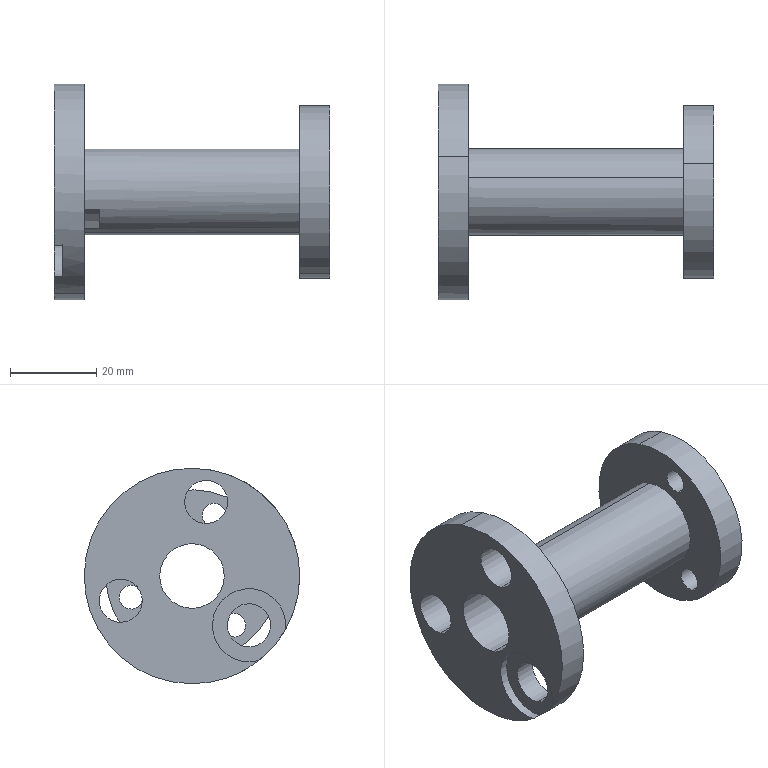Component | SolidWorks | SuctionCupBracket-1 | 1 solid | 29 faces | box 64 x 50 x 50 mm | volume 24493 mm3 | cylinder 23 | plane 6 | commonest cylinder face diameters 10 x6 5.5 x6 17 x3 15 x2 50 x2 40 x2 20 x2
STEP:
#1=COLOUR_RGB('',0.7922,0.8196,0.9333);
#2=FILL_AREA_STYLE_COLOUR('',#1);
#3=FILL_AREA_STYLE('',(#2));
#4=SURFACE_STYLE_FILL_AREA(#3);
#5=SURFACE_SIDE_STYLE('',(#4));
#6=SURFACE_STYLE_USAGE(.BOTH.,#5);
#7=PRESENTATION_STYLE_ASSIGNMENT((#6));
#8=CARTESIAN_POINT('',(-5.854,1.572,-3.839));
#9=VERTEX_POINT('',#8);
#10=CARTESIAN_POINT('',(-5.854,1.375,-4.478));
#11=VERTEX_POINT('',#10);
#12=CARTESIAN_POINT('',(-5.854,1.462,-4.155));
#13=DIRECTION('',(-1.,0.,0.));
#14=DIRECTION('',(0.,0.3282,0.9446));
#15=AXIS2_PLACEMENT_3D('',#12,#13,#14);
#16=CIRCLE('',#15,0.3346);
#17=EDGE_CURVE('',#9,#11,#16,.T.);
#18=ORIENTED_EDGE('',*,*,#17,.F.);
#19=CARTESIAN_POINT('',(-5.933,1.572,-3.839));
#20=VERTEX_POINT('',#19);
#21=CARTESIAN_POINT('',(-5.854,1.572,-3.839));
#22=DIRECTION('',(-1.,0.,0.));
#23=VECTOR('',#22,39.37);
#24=LINE('',#21,#23);
#25=EDGE_CURVE('',#9,#20,#24,.T.);
#26=ORIENTED_EDGE('',*,*,#25,.T.);
#27=CARTESIAN_POINT('',(-5.933,1.375,-4.478));
#28=VERTEX_POINT('',#27);
#29=CARTESIAN_POINT('',(-5.933,1.462,-4.155));
#30=DIRECTION('',(-1.,0.,0.));
#31=DIRECTION('',(0.,0.3282,0.9446));
#32=AXIS2_PLACEMENT_3D('',#29,#30,#31);
#33=CIRCLE('',#32,0.3346);
#34=EDGE_CURVE('',#20,#28,#33,.T.);
#35=ORIENTED_EDGE('',*,*,#34,.T.);
#36=CARTESIAN_POINT('',(-5.893,1.375,-4.478));
#37=DIRECTION('',(-1.,0.,0.));
#38=VECTOR('',#37,39.37);
#39=LINE('',#36,#38);
#40=EDGE_CURVE('',#11,#28,#39,.T.);
#41=ORIENTED_EDGE('',*,*,#40,.F.);
#42=EDGE_LOOP('',(#18,#26,#35,#41));
#43=FACE_OUTER_BOUND('',#42,.T.);
#44=CARTESIAN_POINT('',(-5.854,1.462,-4.155));
#45=DIRECTION('',(-1.,0.,0.));
#46=DIRECTION('',(0.,0.3282,0.9446));
#47=AXIS2_PLACEMENT_3D('',#44,#45,#46);
#48=CYLINDRICAL_SURFACE('',#47,0.3346);
#49=ADVANCED_FACE('',(#43),#48,.F.);
#50=CARTESIAN_POINT('',(-5.657,1.789,-3.214));
#51=VERTEX_POINT('',#50);
#52=CARTESIAN_POINT('',(-5.657,1.919,-2.842));
#53=VERTEX_POINT('',#52);
#54=CARTESIAN_POINT('',(-5.657,1.854,-3.028));
#55=DIRECTION('',(-1.,0.,0.));
#56=DIRECTION('',(0.,-0.9822,-0.1881));
#57=AXIS2_PLACEMENT_3D('',#54,#55,#56);
#58=CIRCLE('',#57,0.1969);
#59=EDGE_CURVE('',#51,#53,#58,.T.);
#60=ORIENTED_EDGE('',*,*,#59,.F.);
#61=CARTESIAN_POINT('',(-5.933,1.789,-3.214));
#62=VERTEX_POINT('',#61);
#63=CARTESIAN_POINT('',(-5.657,1.789,-3.214));
#64=DIRECTION('',(-1.,0.,0.));
#65=VECTOR('',#64,39.37);
#66=LINE('',#63,#65);
#67=EDGE_CURVE('',#51,#62,#66,.T.);
#68=ORIENTED_EDGE('',*,*,#67,.T.);
#69=CARTESIAN_POINT('',(-5.933,1.919,-2.842));
#70=VERTEX_POINT('',#69);
#71=CARTESIAN_POINT('',(-5.933,1.854,-3.028));
#72=DIRECTION('',(-1.,0.,0.));
#73=DIRECTION('',(0.,-0.9822,-0.1881));
#74=AXIS2_PLACEMENT_3D('',#71,#72,#73);
#75=CIRCLE('',#74,0.1969);
#76=EDGE_CURVE('',#62,#70,#75,.T.);
#77=ORIENTED_EDGE('',*,*,#76,.T.);
#78=CARTESIAN_POINT('',(-5.657,1.919,-2.842));
#79=DIRECTION('',(-1.,0.,0.));
#80=VECTOR('',#79,39.37);
#81=LINE('',#78,#80);
#82=EDGE_CURVE('',#53,#70,#81,.T.);
#83=ORIENTED_EDGE('',*,*,#82,.F.);
#84=EDGE_LOOP('',(#60,#68,#77,#83));
#85=FACE_OUTER_BOUND('',#84,.T.);
#86=CARTESIAN_POINT('',(-5.657,1.854,-3.028));
#87=DIRECTION('',(-1.,0.,0.));
#88=DIRECTION('',(0.,0.3282,0.9446));
#89=AXIS2_PLACEMENT_3D('',#86,#87,#88);
#90=CYLINDRICAL_SURFACE('',#89,0.1969);
#91=ADVANCED_FACE('',(#85),#90,.F.);
#92=CARTESIAN_POINT('',(-5.657,2.57,-4.117));
#93=VERTEX_POINT('',#92);
#94=CARTESIAN_POINT('',(-5.657,2.699,-3.745));
#95=VERTEX_POINT('',#94);
#96=CARTESIAN_POINT('',(-5.657,2.634,-3.931));
#97=DIRECTION('',(-1.,0.,0.));
#98=DIRECTION('',(0.,0.3282,0.9446));
#99=AXIS2_PLACEMENT_3D('',#96,#97,#98);
#100=CIRCLE('',#99,0.1969);
#101=EDGE_CURVE('',#93,#95,#100,.T.);
#102=ORIENTED_EDGE('',*,*,#101,.F.);
#103=CARTESIAN_POINT('',(-5.933,2.57,-4.117));
#104=VERTEX_POINT('',#103);
#105=CARTESIAN_POINT('',(-5.657,2.57,-4.117));
#106=DIRECTION('',(-1.,0.,0.));
#107=VECTOR('',#106,39.37);
#108=LINE('',#105,#107);
#109=EDGE_CURVE('',#93,#104,#108,.T.);
#110=ORIENTED_EDGE('',*,*,#109,.T.);
#111=CARTESIAN_POINT('',(-5.933,2.699,-3.745));
#112=VERTEX_POINT('',#111);
#113=CARTESIAN_POINT('',(-5.933,2.634,-3.931));
#114=DIRECTION('',(-1.,0.,0.));
#115=DIRECTION('',(0.,0.3282,0.9446));
#116=AXIS2_PLACEMENT_3D('',#113,#114,#115);
#117=CIRCLE('',#116,0.1969);
#118=EDGE_CURVE('',#104,#112,#117,.T.);
#119=ORIENTED_EDGE('',*,*,#118,.T.);
#120=CARTESIAN_POINT('',(-5.657,2.699,-3.745));
#121=DIRECTION('',(-1.,0.,0.));
#122=VECTOR('',#121,39.37);
#123=LINE('',#120,#122);
#124=EDGE_CURVE('',#95,#112,#123,.T.);
#125=ORIENTED_EDGE('',*,*,#124,.F.);
#126=EDGE_LOOP('',(#102,#110,#119,#125));
#127=FACE_OUTER_BOUND('',#126,.T.);
#128=CARTESIAN_POINT('',(-5.657,2.634,-3.931));
#129=DIRECTION('',(-1.,0.,0.));
#130=DIRECTION('',(0.,0.3282,0.9446));
#131=AXIS2_PLACEMENT_3D('',#128,#129,#130);
#132=CYLINDRICAL_SURFACE('',#131,0.1969);
#133=ADVANCED_FACE('',(#127),#132,.F.);
#134=CARTESIAN_POINT('',(-5.933,2.08,-3.426));
#135=VERTEX_POINT('',#134);
#136=CARTESIAN_POINT('',(-5.933,1.887,-3.983));
#137=VERTEX_POINT('',#136);
#138=CARTESIAN_POINT('',(-5.933,1.983,-3.704));
#139=DIRECTION('',(1.,-0.,-0.));
#140=DIRECTION('',(0.,-0.3282,-0.9446));
#141=AXIS2_PLACEMENT_3D('',#138,#139,#140);
#142=CIRCLE('',#141,0.2953);
#143=EDGE_CURVE('',#135,#137,#142,.T.);
#144=ORIENTED_EDGE('',*,*,#143,.F.);
#145=CARTESIAN_POINT('',(-3.413,2.08,-3.426));
#146=VERTEX_POINT('',#145);
#147=CARTESIAN_POINT('',(-5.933,2.08,-3.426));
#148=DIRECTION('',(1.,-0.,-0.));
#149=VECTOR('',#148,39.37);
#150=LINE('',#147,#149);
#151=EDGE_CURVE('',#135,#146,#150,.T.);
#152=ORIENTED_EDGE('',*,*,#151,.T.);
#153=CARTESIAN_POINT('',(-3.413,1.887,-3.983));
#154=VERTEX_POINT('',#153);
#155=CARTESIAN_POINT('',(-3.413,1.983,-3.704));
#156=DIRECTION('',(1.,-0.,-0.));
#157=DIRECTION('',(0.,-0.3282,-0.9446));
#158=AXIS2_PLACEMENT_3D('',#155,#156,#157);
#159=CIRCLE('',#158,0.2953);
#160=EDGE_CURVE('',#146,#154,#159,.T.);
#161=ORIENTED_EDGE('',*,*,#160,.T.);
#162=CARTESIAN_POINT('',(-5.933,1.887,-3.983));
#163=DIRECTION('',(1.,-0.,-0.));
#164=VECTOR('',#163,39.37);
#165=LINE('',#162,#164);
#166=EDGE_CURVE('',#137,#154,#165,.T.);
#167=ORIENTED_EDGE('',*,*,#166,.F.);
#168=EDGE_LOOP('',(#144,#152,#161,#167));
#169=FACE_OUTER_BOUND('',#168,.T.);
#170=CARTESIAN_POINT('',(-5.933,1.983,-3.704));
#171=DIRECTION('',(1.,-0.,-0.));
#172=DIRECTION('',(0.,-0.3282,-0.9446));
#173=AXIS2_PLACEMENT_3D('',#170,#171,#172);
#174=CYLINDRICAL_SURFACE('',#173,0.2953);
#175=ADVANCED_FACE('',(#169),#174,.F.);
#176=CARTESIAN_POINT('',(-3.689,1.636,-4.052));
#177=VERTEX_POINT('',#176);
#178=CARTESIAN_POINT('',(-3.689,1.565,-4.256));
#179=VERTEX_POINT('',#178);
#180=CARTESIAN_POINT('',(-3.689,1.601,-4.154));
#181=DIRECTION('',(1.,-0.,-0.));
#182=DIRECTION('',(0.,-0.3282,-0.9446));
#183=AXIS2_PLACEMENT_3D('',#180,#181,#182);
#184=CIRCLE('',#183,0.1083);
#185=EDGE_CURVE('',#177,#179,#184,.T.);
#186=ORIENTED_EDGE('',*,*,#185,.F.);
#187=CARTESIAN_POINT('',(-3.413,1.636,-4.052));
#188=VERTEX_POINT('',#187);
#189=CARTESIAN_POINT('',(-3.689,1.636,-4.052));
#190=DIRECTION('',(1.,-0.,-0.));
#191=VECTOR('',#190,39.37);
#192=LINE('',#189,#191);
#193=EDGE_CURVE('',#177,#188,#192,.T.);
#194=ORIENTED_EDGE('',*,*,#193,.T.);
#195=CARTESIAN_POINT('',(-3.413,1.565,-4.256));
#196=VERTEX_POINT('',#195);
#197=CARTESIAN_POINT('',(-3.413,1.601,-4.154));
#198=DIRECTION('',(1.,-0.,-0.));
#199=DIRECTION('',(0.,-0.3282,-0.9446));
#200=AXIS2_PLACEMENT_3D('',#197,#198,#199);
#201=CIRCLE('',#200,0.1083);
#202=EDGE_CURVE('',#188,#196,#201,.T.);
#203=ORIENTED_EDGE('',*,*,#202,.T.);
#204=CARTESIAN_POINT('',(-3.689,1.565,-4.256));
#205=DIRECTION('',(1.,-0.,-0.));
#206=VECTOR('',#205,39.37);
#207=LINE('',#204,#206);
#208=EDGE_CURVE('',#179,#196,#207,.T.);
#209=ORIENTED_EDGE('',*,*,#208,.F.);
#210=EDGE_LOOP('',(#186,#194,#203,#209));
#211=FACE_OUTER_BOUND('',#210,.T.);
#212=CARTESIAN_POINT('',(-3.689,1.601,-4.154));
#213=DIRECTION('',(1.,-0.,-0.));
#214=DIRECTION('',(0.,-0.3282,-0.9446));
#215=AXIS2_PLACEMENT_3D('',#212,#213,#214);
#216=CYLINDRICAL_SURFACE('',#215,0.1083);
#217=ADVANCED_FACE('',(#211),#216,.F.);
#218=CARTESIAN_POINT('',(-3.689,1.819,-3.047));
#219=VERTEX_POINT('',#218);
#220=CARTESIAN_POINT('',(-3.689,1.748,-3.251));
#221=VERTEX_POINT('',#220);
#222=CARTESIAN_POINT('',(-3.689,1.783,-3.149));
#223=DIRECTION('',(1.,-0.,-0.));
#224=DIRECTION('',(0.,-0.3282,-0.9446));
#225=AXIS2_PLACEMENT_3D('',#222,#223,#224);
#226=CIRCLE('',#225,0.1083);
#227=EDGE_CURVE('',#219,#221,#226,.T.);
#228=ORIENTED_EDGE('',*,*,#227,.F.);
#229=CARTESIAN_POINT('',(-3.413,1.819,-3.047));
#230=VERTEX_POINT('',#229);
#231=CARTESIAN_POINT('',(-3.689,1.819,-3.047));
#232=DIRECTION('',(1.,-0.,-0.));
#233=VECTOR('',#232,39.37);
#234=LINE('',#231,#233);
#235=EDGE_CURVE('',#219,#230,#234,.T.);
#236=ORIENTED_EDGE('',*,*,#235,.T.);
#237=CARTESIAN_POINT('',(-3.413,1.748,-3.251));
#238=VERTEX_POINT('',#237);
#239=CARTESIAN_POINT('',(-3.413,1.783,-3.149));
#240=DIRECTION('',(1.,-0.,-0.));
#241=DIRECTION('',(0.,-0.3282,-0.9446));
#242=AXIS2_PLACEMENT_3D('',#239,#240,#241);
#243=CIRCLE('',#242,0.1083);
#244=EDGE_CURVE('',#230,#238,#243,.T.);
#245=ORIENTED_EDGE('',*,*,#244,.T.);
#246=CARTESIAN_POINT('',(-3.689,1.748,-3.251));
#247=DIRECTION('',(1.,-0.,-0.));
#248=VECTOR('',#247,39.37);
#249=LINE('',#246,#248);
#250=EDGE_CURVE('',#221,#238,#249,.T.);
#251=ORIENTED_EDGE('',*,*,#250,.F.);
#252=EDGE_LOOP('',(#228,#236,#245,#251));
#253=FACE_OUTER_BOUND('',#252,.T.);
#254=CARTESIAN_POINT('',(-3.689,1.783,-3.149));
#255=DIRECTION('',(1.,-0.,-0.));
#256=DIRECTION('',(0.,-0.3282,-0.9446));
#257=AXIS2_PLACEMENT_3D('',#254,#255,#256);
#258=CYLINDRICAL_SURFACE('',#257,0.1083);
#259=ADVANCED_FACE('',(#253),#258,.F.);
#260=CARTESIAN_POINT('',(-3.689,2.577,-3.796));
#261=VERTEX_POINT('',#260);
#262=CARTESIAN_POINT('',(-3.689,2.506,-4.001));
#263=VERTEX_POINT('',#262);
#264=CARTESIAN_POINT('',(-3.689,2.541,-3.898));
#265=DIRECTION('',(1.,-0.,-0.));
#266=DIRECTION('',(0.,-0.3282,-0.9446));
#267=AXIS2_PLACEMENT_3D('',#264,#265,#266);
#268=CIRCLE('',#267,0.1083);
#269=EDGE_CURVE('',#261,#263,#268,.T.);
#270=ORIENTED_EDGE('',*,*,#269,.F.);
#271=CARTESIAN_POINT('',(-3.413,2.577,-3.796));
#272=VERTEX_POINT('',#271);
#273=CARTESIAN_POINT('',(-3.689,2.577,-3.796));
#274=DIRECTION('',(1.,-0.,-0.));
#275=VECTOR('',#274,39.37);
#276=LINE('',#273,#275);
#277=EDGE_CURVE('',#261,#272,#276,.T.);
#278=ORIENTED_EDGE('',*,*,#277,.T.);
#279=CARTESIAN_POINT('',(-3.413,2.506,-4.001));
#280=VERTEX_POINT('',#279);
#281=CARTESIAN_POINT('',(-3.413,2.541,-3.898));
#282=DIRECTION('',(1.,-0.,-0.));
#283=DIRECTION('',(0.,-0.3282,-0.9446));
#284=AXIS2_PLACEMENT_3D('',#281,#282,#283);
#285=CIRCLE('',#284,0.1083);
#286=EDGE_CURVE('',#272,#280,#285,.T.);
#287=ORIENTED_EDGE('',*,*,#286,.T.);
#288=CARTESIAN_POINT('',(-3.689,2.506,-4.001));
#289=DIRECTION('',(1.,-0.,-0.));
#290=VECTOR('',#289,39.37);
#291=LINE('',#288,#290);
#292=EDGE_CURVE('',#263,#280,#291,.T.);
#293=ORIENTED_EDGE('',*,*,#292,.F.);
#294=EDGE_LOOP('',(#270,#278,#287,#293));
#295=FACE_OUTER_BOUND('',#294,.T.);
#296=CARTESIAN_POINT('',(-3.689,2.541,-3.898));
#297=DIRECTION('',(1.,-0.,-0.));
#298=DIRECTION('',(0.,-0.3282,-0.9446));
#299=AXIS2_PLACEMENT_3D('',#296,#297,#298);
#300=CYLINDRICAL_SURFACE('',#299,0.1083);
#301=ADVANCED_FACE('',(#295),#300,.F.);
#302=CARTESIAN_POINT('',(-5.933,2.307,-2.775));
#303=VERTEX_POINT('',#302);
#304=CARTESIAN_POINT('',(-5.933,1.66,-4.634));
#305=VERTEX_POINT('',#304);
#306=CARTESIAN_POINT('',(-5.933,1.983,-3.704));
#307=DIRECTION('',(-1.,0.,0.));
#308=DIRECTION('',(0.,0.3282,0.9446));
#309=AXIS2_PLACEMENT_3D('',#306,#307,#308);
#310=CIRCLE('',#309,0.9843);
#311=EDGE_CURVE('',#303,#305,#310,.T.);
#312=ORIENTED_EDGE('',*,*,#311,.F.);
#313=CARTESIAN_POINT('',(-5.657,2.307,-2.775));
#314=VERTEX_POINT('',#313);
#315=CARTESIAN_POINT('',(-5.933,2.307,-2.775));
#316=DIRECTION('',(1.,-0.,-0.));
#317=VECTOR('',#316,39.37);
#318=LINE('',#315,#317);
#319=EDGE_CURVE('',#303,#314,#318,.T.);
#320=ORIENTED_EDGE('',*,*,#319,.T.);
#321=CARTESIAN_POINT('',(-5.657,1.66,-4.634));
#322=VERTEX_POINT('',#321);
#323=CARTESIAN_POINT('',(-5.657,1.983,-3.704));
#324=DIRECTION('',(-1.,0.,0.));
#325=DIRECTION('',(0.,0.3282,0.9446));
#326=AXIS2_PLACEMENT_3D('',#323,#324,#325);
#327=CIRCLE('',#326,0.9843);
#328=EDGE_CURVE('',#314,#322,#327,.T.);
#329=ORIENTED_EDGE('',*,*,#328,.T.);
#330=CARTESIAN_POINT('',(-5.933,1.66,-4.634));
#331=DIRECTION('',(1.,-0.,-0.));
#332=VECTOR('',#331,39.37);
#333=LINE('',#330,#332);
#334=EDGE_CURVE('',#305,#322,#333,.T.);
#335=ORIENTED_EDGE('',*,*,#334,.F.);
#336=EDGE_LOOP('',(#312,#320,#329,#335));
#337=FACE_OUTER_BOUND('',#336,.T.);
#338=CARTESIAN_POINT('',(-5.933,1.983,-3.704));
#339=DIRECTION('',(1.,-0.,-0.));
#340=DIRECTION('',(-0.,-0.3282,-0.9446));
#341=AXIS2_PLACEMENT_3D('',#338,#339,#340);
#342=CYLINDRICAL_SURFACE('',#341,0.9843);
#343=ADVANCED_FACE('',(#337),#342,.T.);
#344=CARTESIAN_POINT('',(-3.413,1.725,-4.448));
#345=VERTEX_POINT('',#344);
#346=CARTESIAN_POINT('',(-3.413,2.242,-2.961));
#347=VERTEX_POINT('',#346);
#348=CARTESIAN_POINT('',(-3.413,1.983,-3.704));
#349=DIRECTION('',(1.,-0.,-0.));
#350=DIRECTION('',(-0.,-0.3282,-0.9446));
#351=AXIS2_PLACEMENT_3D('',#348,#349,#350);
#352=CIRCLE('',#351,0.7874);
#353=EDGE_CURVE('',#345,#347,#352,.T.);
#354=ORIENTED_EDGE('',*,*,#353,.F.);
#355=CARTESIAN_POINT('',(-3.689,1.725,-4.448));
#356=VERTEX_POINT('',#355);
#357=CARTESIAN_POINT('',(-3.413,1.725,-4.448));
#358=DIRECTION('',(-1.,0.,0.));
#359=VECTOR('',#358,39.37);
#360=LINE('',#357,#359);
#361=EDGE_CURVE('',#345,#356,#360,.T.);
#362=ORIENTED_EDGE('',*,*,#361,.T.);
#363=CARTESIAN_POINT('',(-3.689,2.242,-2.961));
#364=VERTEX_POINT('',#363);
#365=CARTESIAN_POINT('',(-3.689,1.983,-3.704));
#366=DIRECTION('',(1.,-0.,-0.));
#367=DIRECTION('',(-0.,-0.3282,-0.9446));
#368=AXIS2_PLACEMENT_3D('',#365,#366,#367);
#369=CIRCLE('',#368,0.7874);
#370=EDGE_CURVE('',#356,#364,#369,.T.);
#371=ORIENTED_EDGE('',*,*,#370,.T.);
#372=CARTESIAN_POINT('',(-3.413,2.242,-2.961));
#373=DIRECTION('',(-1.,0.,0.));
#374=VECTOR('',#373,39.37);
#375=LINE('',#372,#374);
#376=EDGE_CURVE('',#347,#364,#375,.T.);
#377=ORIENTED_EDGE('',*,*,#376,.F.);
#378=EDGE_LOOP('',(#354,#362,#371,#377));
#379=FACE_OUTER_BOUND('',#378,.T.);
#380=CARTESIAN_POINT('',(-3.413,1.983,-3.704));
#381=DIRECTION('',(-1.,0.,0.));
#382=DIRECTION('',(0.,0.3282,0.9446));
#383=AXIS2_PLACEMENT_3D('',#380,#381,#382);
#384=CYLINDRICAL_SURFACE('',#383,0.7874);
#385=ADVANCED_FACE('',(#379),#384,.T.);
#386=CARTESIAN_POINT('',(-5.657,1.398,-4.341));
#387=VERTEX_POINT('',#386);
#388=CARTESIAN_POINT('',(-5.657,1.527,-3.969));
#389=VERTEX_POINT('',#388);
#390=CARTESIAN_POINT('',(-5.657,1.462,-4.155));
#391=DIRECTION('',(-1.,0.,0.));
#392=DIRECTION('',(0.,0.6539,-0.7565));
#393=AXIS2_PLACEMENT_3D('',#390,#391,#392);
#394=CIRCLE('',#393,0.1969);
#395=EDGE_CURVE('',#387,#389,#394,.T.);
#396=ORIENTED_EDGE('',*,*,#395,.F.);
#397=CARTESIAN_POINT('',(-5.854,1.398,-4.341));
#398=VERTEX_POINT('',#397);
#399=CARTESIAN_POINT('',(-5.657,1.398,-4.341));
#400=DIRECTION('',(-1.,0.,0.));
#401=VECTOR('',#400,39.37);
#402=LINE('',#399,#401);
#403=EDGE_CURVE('',#387,#398,#402,.T.);
#404=ORIENTED_EDGE('',*,*,#403,.T.);
#405=CARTESIAN_POINT('',(-5.854,1.527,-3.969));
#406=VERTEX_POINT('',#405);
#407=CARTESIAN_POINT('',(-5.854,1.462,-4.155));
#408=DIRECTION('',(1.,-0.,-0.));
#409=DIRECTION('',(0.,0.3282,0.9446));
#410=AXIS2_PLACEMENT_3D('',#407,#408,#409);
#411=CIRCLE('',#410,0.1969);
#412=EDGE_CURVE('',#406,#398,#411,.T.);
#413=ORIENTED_EDGE('',*,*,#412,.F.);
#414=CARTESIAN_POINT('',(-5.657,1.527,-3.969));
#415=DIRECTION('',(-1.,0.,0.));
#416=VECTOR('',#415,39.37);
#417=LINE('',#414,#416);
#418=EDGE_CURVE('',#389,#406,#417,.T.);
#419=ORIENTED_EDGE('',*,*,#418,.F.);
#420=EDGE_LOOP('',(#396,#404,#413,#419));
#421=FACE_OUTER_BOUND('',#420,.T.);
#422=CARTESIAN_POINT('',(-5.657,1.462,-4.155));
#423=DIRECTION('',(-1.,0.,0.));
#424=DIRECTION('',(0.,0.3282,0.9446));
#425=AXIS2_PLACEMENT_3D('',#422,#423,#424);
#426=CYLINDRICAL_SURFACE('',#425,0.1969);
#427=ADVANCED_FACE('',(#421),#426,.F.);
#428=CARTESIAN_POINT('',(-5.657,2.113,-3.333));
#429=VERTEX_POINT('',#428);
#430=CARTESIAN_POINT('',(-5.657,1.854,-4.076));
#431=VERTEX_POINT('',#430);
#432=CARTESIAN_POINT('',(-5.657,1.983,-3.704));
#433=DIRECTION('',(-1.,0.,0.));
#434=DIRECTION('',(0.,0.3282,0.9446));
#435=AXIS2_PLACEMENT_3D('',#432,#433,#434);
#436=CIRCLE('',#435,0.3937);
#437=EDGE_CURVE('',#429,#431,#436,.T.);
#438=ORIENTED_EDGE('',*,*,#437,.F.);
#439=CARTESIAN_POINT('',(-3.689,2.113,-3.333));
#440=VERTEX_POINT('',#439);
#441=CARTESIAN_POINT('',(-5.657,2.113,-3.333));
#442=DIRECTION('',(1.,-0.,-0.));
#443=VECTOR('',#442,39.37);
#444=LINE('',#441,#443);
#445=EDGE_CURVE('',#429,#440,#444,.T.);
#446=ORIENTED_EDGE('',*,*,#445,.T.);
#447=CARTESIAN_POINT('',(-3.689,1.854,-4.076));
#448=VERTEX_POINT('',#447);
#449=CARTESIAN_POINT('',(-3.689,1.983,-3.704));
#450=DIRECTION('',(-1.,0.,0.));
#451=DIRECTION('',(-0.,-0.3282,-0.9446));
#452=AXIS2_PLACEMENT_3D('',#449,#450,#451);
#453=CIRCLE('',#452,0.3937);
#454=EDGE_CURVE('',#440,#448,#453,.T.);
#455=ORIENTED_EDGE('',*,*,#454,.T.);
#456=CARTESIAN_POINT('',(-5.657,1.854,-4.076));
#457=DIRECTION('',(1.,-0.,-0.));
#458=VECTOR('',#457,39.37);
#459=LINE('',#456,#458);
#460=EDGE_CURVE('',#431,#448,#459,.T.);
#461=ORIENTED_EDGE('',*,*,#460,.F.);
#462=EDGE_LOOP('',(#438,#446,#455,#461));
#463=FACE_OUTER_BOUND('',#462,.T.);
#464=CARTESIAN_POINT('',(-5.657,1.983,-3.704));
#465=DIRECTION('',(1.,-0.,-0.));
#466=DIRECTION('',(0.,-0.3282,-0.9446));
#467=AXIS2_PLACEMENT_3D('',#464,#465,#466);
#468=CYLINDRICAL_SURFACE('',#467,0.3937);
#469=ADVANCED_FACE('',(#463),#468,.T.);
#470=ORIENTED_EDGE('',*,*,#445,.F.);
#471=CARTESIAN_POINT('',(-5.657,1.622,-3.861));
#472=VERTEX_POINT('',#471);
#473=CARTESIAN_POINT('',(-5.657,1.983,-3.704));
#474=DIRECTION('',(-1.,0.,0.));
#475=DIRECTION('',(0.,0.3282,0.9446));
#476=AXIS2_PLACEMENT_3D('',#473,#474,#475);
#477=CIRCLE('',#476,0.3937);
#478=EDGE_CURVE('',#472,#429,#477,.T.);
#479=ORIENTED_EDGE('',*,*,#478,.F.);
#480=CARTESIAN_POINT('',(-5.519,1.622,-3.861));
#481=VERTEX_POINT('',#480);
#482=CARTESIAN_POINT('',(-5.588,1.622,-3.861));
#483=DIRECTION('',(-1.,0.,0.));
#484=VECTOR('',#483,39.37);
#485=LINE('',#482,#484);
#486=EDGE_CURVE('',#481,#472,#485,.T.);
#487=ORIENTED_EDGE('',*,*,#486,.F.);
#488=CARTESIAN_POINT('',(-5.519,1.776,-4.039));
#489=VERTEX_POINT('',#488);
#490=CARTESIAN_POINT('',(-5.519,1.983,-3.704));
#491=DIRECTION('',(1.,-0.,-0.));
#492=DIRECTION('',(0.,-0.3282,-0.9446));
#493=AXIS2_PLACEMENT_3D('',#490,#491,#492);
#494=CIRCLE('',#493,0.3937);
#495=EDGE_CURVE('',#481,#489,#494,.T.);
#496=ORIENTED_EDGE('',*,*,#495,.T.);
#497=CARTESIAN_POINT('',(-5.657,1.776,-4.039));
#498=VERTEX_POINT('',#497);
#499=CARTESIAN_POINT('',(-5.588,1.776,-4.039));
#500=DIRECTION('',(1.,-0.,-0.));
#501=VECTOR('',#500,39.37);
#502=LINE('',#499,#501);
#503=EDGE_CURVE('',#498,#489,#502,.T.);
#504=ORIENTED_EDGE('',*,*,#503,.F.);
#505=CARTESIAN_POINT('',(-5.657,1.983,-3.704));
#506=DIRECTION('',(-1.,0.,0.));
#507=DIRECTION('',(0.,0.3282,0.9446));
#508=AXIS2_PLACEMENT_3D('',#505,#506,#507);
#509=CIRCLE('',#508,0.3937);
#510=EDGE_CURVE('',#431,#498,#509,.T.);
#511=ORIENTED_EDGE('',*,*,#510,.F.);
#512=ORIENTED_EDGE('',*,*,#460,.T.);
#513=CARTESIAN_POINT('',(-3.689,1.983,-3.704));
#514=DIRECTION('',(-1.,0.,0.));
#515=DIRECTION('',(-0.,-0.3282,-0.9446));
#516=AXIS2_PLACEMENT_3D('',#513,#514,#515);
#517=CIRCLE('',#516,0.3937);
#518=EDGE_CURVE('',#448,#440,#517,.T.);
#519=ORIENTED_EDGE('',*,*,#518,.T.);
#520=EDGE_LOOP('',(#470,#479,#487,#496,#504,#511,#512,#519));
#521=FACE_OUTER_BOUND('',#520,.T.);
#522=CARTESIAN_POINT('',(-5.657,1.983,-3.704));
#523=DIRECTION('',(1.,-0.,-0.));
#524=DIRECTION('',(0.,-0.3282,-0.9446));
#525=AXIS2_PLACEMENT_3D('',#522,#523,#524);
#526=CYLINDRICAL_SURFACE('',#525,0.3937);
#527=ADVANCED_FACE('',(#521),#526,.T.);
#528=ORIENTED_EDGE('',*,*,#403,.F.);
#529=CARTESIAN_POINT('',(-5.657,1.462,-4.155));
#530=DIRECTION('',(-1.,0.,0.));
#531=DIRECTION('',(0.,0.6539,-0.7565));
#532=AXIS2_PLACEMENT_3D('',#529,#530,#531);
#533=CIRCLE('',#532,0.1969);
#534=EDGE_CURVE('',#389,#387,#533,.T.);
#535=ORIENTED_EDGE('',*,*,#534,.F.);
#536=ORIENTED_EDGE('',*,*,#418,.T.);
#537=CARTESIAN_POINT('',(-5.854,1.462,-4.155));
#538=DIRECTION('',(1.,-0.,-0.));
#539=DIRECTION('',(0.,0.3282,0.9446));
#540=AXIS2_PLACEMENT_3D('',#537,#538,#539);
#541=CIRCLE('',#540,0.1969);
#542=EDGE_CURVE('',#398,#406,#541,.T.);
#543=ORIENTED_EDGE('',*,*,#542,.F.);
#544=EDGE_LOOP('',(#528,#535,#536,#543));
#545=FACE_OUTER_BOUND('',#544,.T.);
#546=CARTESIAN_POINT('',(-5.657,1.462,-4.155));
#547=DIRECTION('',(-1.,0.,0.));
#548=DIRECTION('',(0.,0.3282,0.9446));
#549=AXIS2_PLACEMENT_3D('',#546,#547,#548);
#550=CYLINDRICAL_SURFACE('',#549,0.1969);
#551=ADVANCED_FACE('',(#545),#550,.F.);
#552=CARTESIAN_POINT('',(-3.689,1.601,-4.154));
#553=DIRECTION('',(1.,-0.,-0.));
#554=DIRECTION('',(0.,-0.3282,-0.9446));
#555=AXIS2_PLACEMENT_3D('',#552,#553,#554);
#556=CIRCLE('',#555,0.1083);
#557=EDGE_CURVE('',#179,#177,#556,.T.);
#558=ORIENTED_EDGE('',*,*,#557,.T.);
#559=ORIENTED_EDGE('',*,*,#185,.T.);
#560=EDGE_LOOP('',(#558,#559));
#561=FACE_BOUND('',#560,.T.);
#562=CARTESIAN_POINT('',(-3.689,1.783,-3.149));
#563=DIRECTION('',(1.,-0.,-0.));
#564=DIRECTION('',(0.,-0.3282,-0.9446));
#565=AXIS2_PLACEMENT_3D('',#562,#563,#564);
#566=CIRCLE('',#565,0.1083);
#567=EDGE_CURVE('',#221,#219,#566,.T.);
#568=ORIENTED_EDGE('',*,*,#567,.T.);
#569=ORIENTED_EDGE('',*,*,#227,.T.);
#570=EDGE_LOOP('',(#568,#569));
#571=FACE_BOUND('',#570,.T.);
#572=CARTESIAN_POINT('',(-3.689,2.541,-3.898));
#573=DIRECTION('',(1.,-0.,-0.));
#574=DIRECTION('',(0.,-0.3282,-0.9446));
#575=AXIS2_PLACEMENT_3D('',#572,#573,#574);
#576=CIRCLE('',#575,0.1083);
#577=EDGE_CURVE('',#263,#261,#576,.T.);
#578=ORIENTED_EDGE('',*,*,#577,.T.);
#579=ORIENTED_EDGE('',*,*,#269,.T.);
#580=EDGE_LOOP('',(#578,#579));
#581=FACE_BOUND('',#580,.T.);
#582=CARTESIAN_POINT('',(-3.689,1.983,-3.704));
#583=DIRECTION('',(1.,-0.,-0.));
#584=DIRECTION('',(-0.,-0.3282,-0.9446));
#585=AXIS2_PLACEMENT_3D('',#582,#583,#584);
#586=CIRCLE('',#585,0.7874);
#587=EDGE_CURVE('',#364,#356,#586,.T.);
#588=ORIENTED_EDGE('',*,*,#587,.F.);
#589=ORIENTED_EDGE('',*,*,#370,.F.);
#590=EDGE_LOOP('',(#588,#589));
#591=FACE_OUTER_BOUND('',#590,.T.);
#592=ORIENTED_EDGE('',*,*,#518,.F.);
#593=ORIENTED_EDGE('',*,*,#454,.F.);
#594=EDGE_LOOP('',(#592,#593));
#595=FACE_BOUND('',#594,.T.);
#596=CARTESIAN_POINT('',(-3.689,1.983,-3.704));
#597=DIRECTION('',(1.,-0.,-0.));
#598=DIRECTION('',(-0.,-0.3282,-0.9446));
#599=AXIS2_PLACEMENT_3D('',#596,#597,#598);
#600=PLANE('',#599);
#601=ADVANCED_FACE('',(#561,#571,#581,#591,#595),#600,.F.);
#602=ORIENTED_EDGE('',*,*,#361,.F.);
#603=CARTESIAN_POINT('',(-3.413,1.983,-3.704));
#604=DIRECTION('',(1.,-0.,-0.));
#605=DIRECTION('',(-0.,-0.3282,-0.9446));
#606=AXIS2_PLACEMENT_3D('',#603,#604,#605);
#607=CIRCLE('',#606,0.7874);
#608=EDGE_CURVE('',#347,#345,#607,.T.);
#609=ORIENTED_EDGE('',*,*,#608,.F.);
#610=ORIENTED_EDGE('',*,*,#376,.T.);
#611=ORIENTED_EDGE('',*,*,#587,.T.);
#612=EDGE_LOOP('',(#602,#609,#610,#611));
#613=FACE_OUTER_BOUND('',#612,.T.);
#614=CARTESIAN_POINT('',(-3.413,1.983,-3.704));
#615=DIRECTION('',(-1.,0.,0.));
#616=DIRECTION('',(0.,0.3282,0.9446));
#617=AXIS2_PLACEMENT_3D('',#614,#615,#616);
#618=CYLINDRICAL_SURFACE('',#617,0.7874);
#619=ADVANCED_FACE('',(#613),#618,.T.);
#620=CARTESIAN_POINT('',(-3.413,1.983,-3.704));
#621=DIRECTION('',(1.,-0.,-0.));
#622=DIRECTION('',(0.,-0.3282,-0.9446));
#623=AXIS2_PLACEMENT_3D('',#620,#621,#622);
#624=CIRCLE('',#623,0.2953);
#625=EDGE_CURVE('',#154,#146,#624,.T.);
#626=ORIENTED_EDGE('',*,*,#625,.F.);
#627=ORIENTED_EDGE('',*,*,#160,.F.);
#628=EDGE_LOOP('',(#626,#627));
#629=FACE_BOUND('',#628,.T.);
#630=CARTESIAN_POINT('',(-3.413,1.601,-4.154));
#631=DIRECTION('',(1.,-0.,-0.));
#632=DIRECTION('',(0.,-0.3282,-0.9446));
#633=AXIS2_PLACEMENT_3D('',#630,#631,#632);
#634=CIRCLE('',#633,0.1083);
#635=EDGE_CURVE('',#196,#188,#634,.T.);
#636=ORIENTED_EDGE('',*,*,#635,.F.);
#637=ORIENTED_EDGE('',*,*,#202,.F.);
#638=EDGE_LOOP('',(#636,#637));
#639=FACE_BOUND('',#638,.T.);
#640=CARTESIAN_POINT('',(-3.413,1.783,-3.149));
#641=DIRECTION('',(1.,-0.,-0.));
#642=DIRECTION('',(0.,-0.3282,-0.9446));
#643=AXIS2_PLACEMENT_3D('',#640,#641,#642);
#644=CIRCLE('',#643,0.1083);
#645=EDGE_CURVE('',#238,#230,#644,.T.);
#646=ORIENTED_EDGE('',*,*,#645,.F.);
#647=ORIENTED_EDGE('',*,*,#244,.F.);
#648=EDGE_LOOP('',(#646,#647));
#649=FACE_BOUND('',#648,.T.);
#650=CARTESIAN_POINT('',(-3.413,2.541,-3.898));
#651=DIRECTION('',(1.,-0.,-0.));
#652=DIRECTION('',(0.,-0.3282,-0.9446));
#653=AXIS2_PLACEMENT_3D('',#650,#651,#652);
#654=CIRCLE('',#653,0.1083);
#655=EDGE_CURVE('',#280,#272,#654,.T.);
#656=ORIENTED_EDGE('',*,*,#655,.F.);
#657=ORIENTED_EDGE('',*,*,#286,.F.);
#658=EDGE_LOOP('',(#656,#657));
#659=FACE_BOUND('',#658,.T.);
#660=ORIENTED_EDGE('',*,*,#608,.T.);
#661=ORIENTED_EDGE('',*,*,#353,.T.);
#662=EDGE_LOOP('',(#660,#661));
#663=FACE_OUTER_BOUND('',#662,.T.);
#664=CARTESIAN_POINT('',(-3.413,1.983,-3.704));
#665=DIRECTION('',(1.,-0.,-0.));
#666=DIRECTION('',(-0.,-0.3282,-0.9446));
#667=AXIS2_PLACEMENT_3D('',#664,#665,#666);
#668=PLANE('',#667);
#669=ADVANCED_FACE('',(#629,#639,#649,#659,#663),#668,.T.);
#670=ORIENTED_EDGE('',*,*,#478,.T.);
#671=ORIENTED_EDGE('',*,*,#437,.T.);
#672=ORIENTED_EDGE('',*,*,#510,.T.);
#673=CARTESIAN_POINT('',(-5.657,1.462,-4.155));
#674=DIRECTION('',(1.,-0.,-0.));
#675=DIRECTION('',(0.,-0.3282,-0.9446));
#676=AXIS2_PLACEMENT_3D('',#673,#674,#675);
#677=CIRCLE('',#676,0.3346);
#678=EDGE_CURVE('',#498,#472,#677,.T.);
#679=ORIENTED_EDGE('',*,*,#678,.T.);
#680=EDGE_LOOP('',(#670,#671,#672,#679));
#681=FACE_BOUND('',#680,.T.);
#682=CARTESIAN_POINT('',(-5.657,1.983,-3.704));
#683=DIRECTION('',(-1.,0.,0.));
#684=DIRECTION('',(0.,0.3282,0.9446));
#685=AXIS2_PLACEMENT_3D('',#682,#683,#684);
#686=CIRCLE('',#685,0.9843);
#687=EDGE_CURVE('',#322,#314,#686,.T.);
#688=ORIENTED_EDGE('',*,*,#687,.F.);
#689=ORIENTED_EDGE('',*,*,#328,.F.);
#690=EDGE_LOOP('',(#688,#689));
#691=FACE_OUTER_BOUND('',#690,.T.);
#692=CARTESIAN_POINT('',(-5.657,1.854,-3.028));
#693=DIRECTION('',(-1.,0.,0.));
#694=DIRECTION('',(0.,-0.9822,-0.1881));
#695=AXIS2_PLACEMENT_3D('',#692,#693,#694);
#696=CIRCLE('',#695,0.1969);
#697=EDGE_CURVE('',#53,#51,#696,.T.);
#698=ORIENTED_EDGE('',*,*,#697,.T.);
#699=ORIENTED_EDGE('',*,*,#59,.T.);
#700=EDGE_LOOP('',(#698,#699));
#701=FACE_BOUND('',#700,.T.);
#702=CARTESIAN_POINT('',(-5.657,2.634,-3.931));
#703=DIRECTION('',(-1.,0.,0.));
#704=DIRECTION('',(0.,0.3282,0.9446));
#705=AXIS2_PLACEMENT_3D('',#702,#703,#704);
#706=CIRCLE('',#705,0.1969);
#707=EDGE_CURVE('',#95,#93,#706,.T.);
#708=ORIENTED_EDGE('',*,*,#707,.T.);
#709=ORIENTED_EDGE('',*,*,#101,.T.);
#710=EDGE_LOOP('',(#708,#709));
#711=FACE_BOUND('',#710,.T.);
#712=ORIENTED_EDGE('',*,*,#534,.T.);
#713=ORIENTED_EDGE('',*,*,#395,.T.);
#714=EDGE_LOOP('',(#712,#713));
#715=FACE_BOUND('',#714,.T.);
#716=CARTESIAN_POINT('',(-5.657,1.983,-3.704));
#717=DIRECTION('',(-1.,0.,0.));
#718=DIRECTION('',(0.,0.3282,0.9446));
#719=AXIS2_PLACEMENT_3D('',#716,#717,#718);
#720=PLANE('',#719);
#721=ADVANCED_FACE('',(#681,#691,#701,#711,#715),#720,.F.);
#722=ORIENTED_EDGE('',*,*,#319,.F.);
#723=CARTESIAN_POINT('',(-5.933,1.13,-4.195));
#724=VERTEX_POINT('',#723);
#725=CARTESIAN_POINT('',(-5.933,1.983,-3.704));
#726=DIRECTION('',(-1.,0.,0.));
#727=DIRECTION('',(0.,0.3282,0.9446));
#728=AXIS2_PLACEMENT_3D('',#725,#726,#727);
#729=CIRCLE('',#728,0.9843);
#730=EDGE_CURVE('',#724,#303,#729,.T.);
#731=ORIENTED_EDGE('',*,*,#730,.F.);
#732=CARTESIAN_POINT('',(-5.854,1.13,-4.195));
#733=VERTEX_POINT('',#732);
#734=CARTESIAN_POINT('',(-5.893,1.13,-4.195));
#735=DIRECTION('',(1.,-0.,-0.));
#736=VECTOR('',#735,39.37);
#737=LINE('',#734,#736);
#738=EDGE_CURVE('',#724,#733,#737,.T.);
#739=ORIENTED_EDGE('',*,*,#738,.T.);
#740=CARTESIAN_POINT('',(-5.854,1.983,-3.704));
#741=DIRECTION('',(-1.,0.,0.));
#742=DIRECTION('',(0.,0.3282,0.9446));
#743=AXIS2_PLACEMENT_3D('',#740,#741,#742);
#744=CIRCLE('',#743,0.9843);
#745=EDGE_CURVE('',#11,#733,#744,.T.);
#746=ORIENTED_EDGE('',*,*,#745,.F.);
#747=ORIENTED_EDGE('',*,*,#40,.T.);
#748=CARTESIAN_POINT('',(-5.933,1.983,-3.704));
#749=DIRECTION('',(-1.,0.,0.));
#750=DIRECTION('',(0.,0.3282,0.9446));
#751=AXIS2_PLACEMENT_3D('',#748,#749,#750);
#752=CIRCLE('',#751,0.9843);
#753=EDGE_CURVE('',#305,#28,#752,.T.);
#754=ORIENTED_EDGE('',*,*,#753,.F.);
#755=ORIENTED_EDGE('',*,*,#334,.T.);
#756=ORIENTED_EDGE('',*,*,#687,.T.);
#757=EDGE_LOOP('',(#722,#731,#739,#746,#747,#754,#755,#756));
#758=FACE_OUTER_BOUND('',#757,.T.);
#759=CARTESIAN_POINT('',(-5.933,1.983,-3.704));
#760=DIRECTION('',(1.,-0.,-0.));
#761=DIRECTION('',(-0.,-0.3282,-0.9446));
#762=AXIS2_PLACEMENT_3D('',#759,#760,#761);
#763=CYLINDRICAL_SURFACE('',#762,0.9843);
#764=ADVANCED_FACE('',(#758),#763,.T.);
#765=CARTESIAN_POINT('',(-5.933,1.462,-4.155));
#766=DIRECTION('',(-1.,0.,0.));
#767=DIRECTION('',(0.,0.3282,0.9446));
#768=AXIS2_PLACEMENT_3D('',#765,#766,#767);
#769=CIRCLE('',#768,0.3346);
#770=EDGE_CURVE('',#724,#20,#769,.T.);
#771=ORIENTED_EDGE('',*,*,#770,.F.);
#772=ORIENTED_EDGE('',*,*,#730,.T.);
#773=ORIENTED_EDGE('',*,*,#311,.T.);
#774=ORIENTED_EDGE('',*,*,#753,.T.);
#775=ORIENTED_EDGE('',*,*,#34,.F.);
#776=EDGE_LOOP('',(#771,#772,#773,#774,#775));
#777=FACE_OUTER_BOUND('',#776,.T.);
#778=CARTESIAN_POINT('',(-5.933,1.854,-3.028));
#779=DIRECTION('',(-1.,0.,0.));
#780=DIRECTION('',(0.,-0.9822,-0.1881));
#781=AXIS2_PLACEMENT_3D('',#778,#779,#780);
#782=CIRCLE('',#781,0.1969);
#783=EDGE_CURVE('',#70,#62,#782,.T.);
#784=ORIENTED_EDGE('',*,*,#783,.F.);
#785=ORIENTED_EDGE('',*,*,#76,.F.);
#786=EDGE_LOOP('',(#784,#785));
#787=FACE_BOUND('',#786,.T.);
#788=CARTESIAN_POINT('',(-5.933,2.634,-3.931));
#789=DIRECTION('',(-1.,0.,0.));
#790=DIRECTION('',(0.,0.3282,0.9446));
#791=AXIS2_PLACEMENT_3D('',#788,#789,#790);
#792=CIRCLE('',#791,0.1969);
#793=EDGE_CURVE('',#112,#104,#792,.T.);
#794=ORIENTED_EDGE('',*,*,#793,.F.);
#795=ORIENTED_EDGE('',*,*,#118,.F.);
#796=EDGE_LOOP('',(#794,#795));
#797=FACE_BOUND('',#796,.T.);
#798=CARTESIAN_POINT('',(-5.933,1.983,-3.704));
#799=DIRECTION('',(1.,-0.,-0.));
#800=DIRECTION('',(0.,-0.3282,-0.9446));
#801=AXIS2_PLACEMENT_3D('',#798,#799,#800);
#802=CIRCLE('',#801,0.2953);
#803=EDGE_CURVE('',#137,#135,#802,.T.);
#804=ORIENTED_EDGE('',*,*,#803,.T.);
#805=ORIENTED_EDGE('',*,*,#143,.T.);
#806=EDGE_LOOP('',(#804,#805));
#807=FACE_BOUND('',#806,.T.);
#808=CARTESIAN_POINT('',(-5.933,1.983,-3.704));
#809=DIRECTION('',(-1.,0.,0.));
#810=DIRECTION('',(0.,0.3282,0.9446));
#811=AXIS2_PLACEMENT_3D('',#808,#809,#810);
#812=PLANE('',#811);
#813=ADVANCED_FACE('',(#777,#787,#797,#807),#812,.T.);
#814=ORIENTED_EDGE('',*,*,#277,.F.);
#815=ORIENTED_EDGE('',*,*,#577,.F.);
#816=ORIENTED_EDGE('',*,*,#292,.T.);
#817=ORIENTED_EDGE('',*,*,#655,.T.);
#818=EDGE_LOOP('',(#814,#815,#816,#817));
#819=FACE_OUTER_BOUND('',#818,.T.);
#820=CARTESIAN_POINT('',(-3.689,2.541,-3.898));
#821=DIRECTION('',(1.,-0.,-0.));
#822=DIRECTION('',(0.,-0.3282,-0.9446));
#823=AXIS2_PLACEMENT_3D('',#820,#821,#822);
#824=CYLINDRICAL_SURFACE('',#823,0.1083);
#825=ADVANCED_FACE('',(#819),#824,.F.);
#826=ORIENTED_EDGE('',*,*,#235,.F.);
#827=ORIENTED_EDGE('',*,*,#567,.F.);
#828=ORIENTED_EDGE('',*,*,#250,.T.);
#829=ORIENTED_EDGE('',*,*,#645,.T.);
#830=EDGE_LOOP('',(#826,#827,#828,#829));
#831=FACE_OUTER_BOUND('',#830,.T.);
#832=CARTESIAN_POINT('',(-3.689,1.783,-3.149));
#833=DIRECTION('',(1.,-0.,-0.));
#834=DIRECTION('',(0.,-0.3282,-0.9446));
#835=AXIS2_PLACEMENT_3D('',#832,#833,#834);
#836=CYLINDRICAL_SURFACE('',#835,0.1083);
#837=ADVANCED_FACE('',(#831),#836,.F.);
#838=ORIENTED_EDGE('',*,*,#193,.F.);
#839=ORIENTED_EDGE('',*,*,#557,.F.);
#840=ORIENTED_EDGE('',*,*,#208,.T.);
#841=ORIENTED_EDGE('',*,*,#635,.T.);
#842=EDGE_LOOP('',(#838,#839,#840,#841));
#843=FACE_OUTER_BOUND('',#842,.T.);
#844=CARTESIAN_POINT('',(-3.689,1.601,-4.154));
#845=DIRECTION('',(1.,-0.,-0.));
#846=DIRECTION('',(0.,-0.3282,-0.9446));
#847=AXIS2_PLACEMENT_3D('',#844,#845,#846);
#848=CYLINDRICAL_SURFACE('',#847,0.1083);
#849=ADVANCED_FACE('',(#843),#848,.F.);
#850=ORIENTED_EDGE('',*,*,#151,.F.);
#851=ORIENTED_EDGE('',*,*,#803,.F.);
#852=ORIENTED_EDGE('',*,*,#166,.T.);
#853=ORIENTED_EDGE('',*,*,#625,.T.);
#854=EDGE_LOOP('',(#850,#851,#852,#853));
#855=FACE_OUTER_BOUND('',#854,.T.);
#856=CARTESIAN_POINT('',(-5.933,1.983,-3.704));
#857=DIRECTION('',(1.,-0.,-0.));
#858=DIRECTION('',(0.,-0.3282,-0.9446));
#859=AXIS2_PLACEMENT_3D('',#856,#857,#858);
#860=CYLINDRICAL_SURFACE('',#859,0.2953);
#861=ADVANCED_FACE('',(#855),#860,.F.);
#862=ORIENTED_EDGE('',*,*,#109,.F.);
#863=ORIENTED_EDGE('',*,*,#707,.F.);
#864=ORIENTED_EDGE('',*,*,#124,.T.);
#865=ORIENTED_EDGE('',*,*,#793,.T.);
#866=EDGE_LOOP('',(#862,#863,#864,#865));
#867=FACE_OUTER_BOUND('',#866,.T.);
#868=CARTESIAN_POINT('',(-5.657,2.634,-3.931));
#869=DIRECTION('',(-1.,0.,0.));
#870=DIRECTION('',(0.,0.3282,0.9446));
#871=AXIS2_PLACEMENT_3D('',#868,#869,#870);
#872=CYLINDRICAL_SURFACE('',#871,0.1969);
#873=ADVANCED_FACE('',(#867),#872,.F.);
#874=ORIENTED_EDGE('',*,*,#67,.F.);
#875=ORIENTED_EDGE('',*,*,#697,.F.);
#876=ORIENTED_EDGE('',*,*,#82,.T.);
#877=ORIENTED_EDGE('',*,*,#783,.T.);
#878=EDGE_LOOP('',(#874,#875,#876,#877));
#879=FACE_OUTER_BOUND('',#878,.T.);
#880=CARTESIAN_POINT('',(-5.657,1.854,-3.028));
#881=DIRECTION('',(-1.,0.,0.));
#882=DIRECTION('',(0.,0.3282,0.9446));
#883=AXIS2_PLACEMENT_3D('',#880,#881,#882);
#884=CYLINDRICAL_SURFACE('',#883,0.1969);
#885=ADVANCED_FACE('',(#879),#884,.F.);
#886=ORIENTED_EDGE('',*,*,#25,.F.);
#887=CARTESIAN_POINT('',(-5.854,1.462,-4.155));
#888=DIRECTION('',(-1.,0.,0.));
#889=DIRECTION('',(0.,0.3282,0.9446));
#890=AXIS2_PLACEMENT_3D('',#887,#888,#889);
#891=CIRCLE('',#890,0.3346);
#892=EDGE_CURVE('',#733,#9,#891,.T.);
#893=ORIENTED_EDGE('',*,*,#892,.F.);
#894=ORIENTED_EDGE('',*,*,#738,.F.);
#895=ORIENTED_EDGE('',*,*,#770,.T.);
#896=EDGE_LOOP('',(#886,#893,#894,#895));
#897=FACE_OUTER_BOUND('',#896,.T.);
#898=CARTESIAN_POINT('',(-5.854,1.462,-4.155));
#899=DIRECTION('',(-1.,0.,0.));
#900=DIRECTION('',(0.,0.3282,0.9446));
#901=AXIS2_PLACEMENT_3D('',#898,#899,#900);
#902=CYLINDRICAL_SURFACE('',#901,0.3346);
#903=ADVANCED_FACE('',(#897),#902,.F.);
#904=ORIENTED_EDGE('',*,*,#412,.T.);
#905=ORIENTED_EDGE('',*,*,#542,.T.);
#906=EDGE_LOOP('',(#904,#905));
#907=FACE_BOUND('',#906,.T.);
#908=ORIENTED_EDGE('',*,*,#745,.T.);
#909=ORIENTED_EDGE('',*,*,#892,.T.);
#910=ORIENTED_EDGE('',*,*,#17,.T.);
#911=EDGE_LOOP('',(#908,#909,#910));
#912=FACE_OUTER_BOUND('',#911,.T.);
#913=CARTESIAN_POINT('',(-5.854,1.462,-4.155));
#914=DIRECTION('',(-1.,0.,0.));
#915=DIRECTION('',(0.,0.3282,0.9446));
#916=AXIS2_PLACEMENT_3D('',#913,#914,#915);
#917=PLANE('',#916);
#918=ADVANCED_FACE('',(#907,#912),#917,.T.);
#919=CARTESIAN_POINT('',(-5.519,1.462,-4.155));
#920=DIRECTION('',(1.,-0.,-0.));
#921=DIRECTION('',(0.,-0.3282,-0.9446));
#922=AXIS2_PLACEMENT_3D('',#919,#920,#921);
#923=CIRCLE('',#922,0.3346);
#924=EDGE_CURVE('',#489,#481,#923,.T.);
#925=ORIENTED_EDGE('',*,*,#924,.F.);
#926=ORIENTED_EDGE('',*,*,#495,.F.);
#927=EDGE_LOOP('',(#925,#926));
#928=FACE_OUTER_BOUND('',#927,.T.);
#929=CARTESIAN_POINT('',(-5.519,1.462,-4.155));
#930=DIRECTION('',(1.,-0.,-0.));
#931=DIRECTION('',(-0.,-0.3282,-0.9446));
#932=AXIS2_PLACEMENT_3D('',#929,#930,#931);
#933=PLANE('',#932);
#934=ADVANCED_FACE('',(#928),#933,.F.);
#935=ORIENTED_EDGE('',*,*,#503,.T.);
#936=ORIENTED_EDGE('',*,*,#924,.T.);
#937=ORIENTED_EDGE('',*,*,#486,.T.);
#938=ORIENTED_EDGE('',*,*,#678,.F.);
#939=EDGE_LOOP('',(#935,#936,#937,#938));
#940=FACE_OUTER_BOUND('',#939,.T.);
#941=CARTESIAN_POINT('',(-5.519,1.462,-4.155));
#942=DIRECTION('',(-1.,0.,0.));
#943=DIRECTION('',(0.,0.3282,0.9446));
#944=AXIS2_PLACEMENT_3D('',#941,#942,#943);
#945=CYLINDRICAL_SURFACE('',#944,0.3346);
#946=ADVANCED_FACE('',(#940),#945,.F.);
#947=CLOSED_SHELL('',(#49,#91,#133,#175,#217,#259,#301,#343,#385,#427,#469,#527,#551,#601,#619,#669,#721,#764,#813,#825,#837,#849,#861,#873,#885,#903,#918,#934,#946));
#948=MANIFOLD_SOLID_BREP('',#947);
#949=STYLED_ITEM('',(#7),#948);
#950=(LENGTH_UNIT()NAMED_UNIT(*)SI_UNIT($,.METRE.));
#951=LENGTH_MEASURE_WITH_UNIT(LENGTH_MEASURE(0.0254),#950);
#952=DIMENSIONAL_EXPONENTS(1.,0.,0.,0.,0.,0.,0.);
#953=(CONVERSION_BASED_UNIT('',#951)LENGTH_UNIT()NAMED_UNIT(#952));
#954=UNCERTAINTY_MEASURE_WITH_UNIT(LENGTH_MEASURE(0.00001),#953,'','');
#955=(NAMED_UNIT(*)PLANE_ANGLE_UNIT()SI_UNIT($,.RADIAN.));
#956=(NAMED_UNIT(*)SI_UNIT($,.STERADIAN.)SOLID_ANGLE_UNIT());
#957=(GEOMETRIC_REPRESENTATION_CONTEXT(3)GLOBAL_UNCERTAINTY_ASSIGNED_CONTEXT((#954))GLOBAL_UNIT_ASSIGNED_CONTEXT((#953,#955,#956))REPRESENTATION_CONTEXT('',''));
#958=MECHANICAL_DESIGN_GEOMETRIC_PRESENTATION_REPRESENTATION('',(#949),#957);
#959=CARTESIAN_POINT('',(0.,0.,0.));
#960=DIRECTION('',(0.,0.,1.));
#961=DIRECTION('',(1.,0.,0.));
#962=AXIS2_PLACEMENT_3D('',#959,#960,#961);
#963=(LENGTH_UNIT()NAMED_UNIT(*)SI_UNIT($,.METRE.));
#964=LENGTH_MEASURE_WITH_UNIT(LENGTH_MEASURE(0.0254),#963);
#965=DIMENSIONAL_EXPONENTS(1.,0.,0.,0.,0.,0.,0.);
#966=(CONVERSION_BASED_UNIT('',#964)LENGTH_UNIT()NAMED_UNIT(#965));
#967=UNCERTAINTY_MEASURE_WITH_UNIT(LENGTH_MEASURE(0.00001),#966,'','');
#968=(NAMED_UNIT(*)PLANE_ANGLE_UNIT()SI_UNIT($,.RADIAN.));
#969=(NAMED_UNIT(*)SI_UNIT($,.STERADIAN.)SOLID_ANGLE_UNIT());
#970=(GEOMETRIC_REPRESENTATION_CONTEXT(3)GLOBAL_UNCERTAINTY_ASSIGNED_CONTEXT((#967))GLOBAL_UNIT_ASSIGNED_CONTEXT((#966,#968,#969))REPRESENTATION_CONTEXT('',''));
#971=ADVANCED_BREP_SHAPE_REPRESENTATION('',(#948,#962),#970);
#972=PRESENTATION_LAYER_ASSIGNMENT('','',(#949));